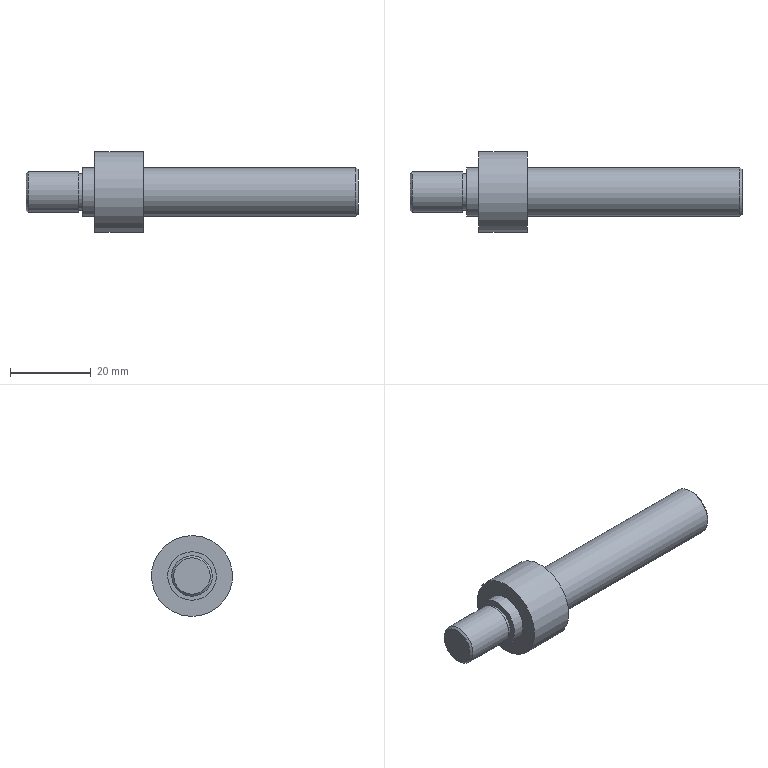Component | NX | SPINDLE | 1 solid | 13 faces | box 82 x 20 x 20 mm | volume 11180 mm3 | plane 6 | cylinder 5 | cone 2 | commonest cylinder face diameters 12 x2 20 x1 9 x1 10 x1
STEP:
#1=CARTESIAN_POINT('',(0.,0.,0.));
#2=DIRECTION('',(0.,0.,1.));
#3=DIRECTION('',(1.,0.,0.));
#4=AXIS2_PLACEMENT_3D('',#1,#2,#3);
#5=CARTESIAN_POINT('',(33.,5.083,38.6));
#6=VERTEX_POINT('',#5);
#7=CARTESIAN_POINT('',(33.,0.,36.5));
#8=DIRECTION('',(1.,0.,0.));
#9=DIRECTION('',(0.,0.9242,0.3818));
#10=AXIS2_PLACEMENT_3D('',#7,#8,#9);
#11=CIRCLE('',#10,5.5);
#12=CARTESIAN_POINT('',(33.,-5.545,34.209));
#13=DIRECTION('',(-1.,0.,0.));
#14=DIRECTION('',(0.,0.9242,0.3818));
#15=AXIS2_PLACEMENT_3D('',#12,#13,#14);
#16=PLANE('',#15);
#17=CARTESIAN_POINT('',(11.5,-0.));
#18=CARTESIAN_POINT('',(11.5,-9.526));
#19=CARTESIAN_POINT('',(3.25,-4.763));
#20=CARTESIAN_POINT('',(-5.,-0.));
#21=CARTESIAN_POINT('',(3.25,4.763));
#22=CARTESIAN_POINT('',(11.5,9.526));
#23=CARTESIAN_POINT('',(11.5,-0.));
#24=(BOUNDED_CURVE()B_SPLINE_CURVE(2,(#17,#18,#19,#20,#21,#22,#23),.UNSPECIFIED.,.T.,.F.)B_SPLINE_CURVE_WITH_KNOTS((1,2,2,2,2,1),(-2.094,0.,2.094,4.189,6.283,8.378),.UNSPECIFIED.)CURVE()GEOMETRIC_REPRESENTATION_ITEM()RATIONAL_B_SPLINE_CURVE((1.,0.5,1.,0.5,1.,0.5,1.))REPRESENTATION_ITEM(''));
#25=(GEOMETRIC_REPRESENTATION_CONTEXT(2)PARAMETRIC_REPRESENTATION_CONTEXT()REPRESENTATION_CONTEXT('',''));
#26=DEFINITIONAL_REPRESENTATION('',(#24),#25);
#27=PCURVE('',#16,#26);
#28=CARTESIAN_POINT('',(33.,0.,36.5));
#29=DIRECTION('',(-1.,0.,0.));
#30=DIRECTION('',(0.,0.9242,0.3818));
#31=AXIS2_PLACEMENT_3D('',#28,#29,#30);
#32=CONICAL_SURFACE('',#31,5.5,0.7854);
#33=CARTESIAN_POINT('',(6.283,-0.));
#34=DIRECTION('',(-1.,0.));
#35=VECTOR('',#34,1.);
#36=LINE('',#33,#35);
#37=(GEOMETRIC_REPRESENTATION_CONTEXT(2)PARAMETRIC_REPRESENTATION_CONTEXT()REPRESENTATION_CONTEXT('',''));
#38=DEFINITIONAL_REPRESENTATION('',(#36),#37);
#39=PCURVE('',#32,#38);
#40=SURFACE_CURVE('',#11,(#27,#39),.PCURVE_S1.);
#41=EDGE_CURVE('',#6,#6,#40,.T.);
#42=ORIENTED_EDGE('',*,*,#41,.T.);
#43=EDGE_LOOP('',(#42));
#44=FACE_BOUND('',#43,.T.);
#45=ADVANCED_FACE('',(#44),#16,.F.);
#46=CARTESIAN_POINT('',(32.5,5.545,38.791));
#47=VERTEX_POINT('',#46);
#48=CARTESIAN_POINT('',(32.5,-5.545,34.209));
#49=VERTEX_POINT('',#48);
#50=CARTESIAN_POINT('',(32.5,0.,36.5));
#51=DIRECTION('',(-1.,0.,0.));
#52=DIRECTION('',(0.,0.9242,0.3818));
#53=AXIS2_PLACEMENT_3D('',#50,#51,#52);
#54=CIRCLE('',#53,6.);
#55=CARTESIAN_POINT('',(33.,0.,36.5));
#56=DIRECTION('',(1.,0.,0.));
#57=DIRECTION('',(0.,-0.9242,-0.3818));
#58=AXIS2_PLACEMENT_3D('',#55,#56,#57);
#59=CYLINDRICAL_SURFACE('',#58,6.);
#60=CARTESIAN_POINT('',(3.142,-0.5));
#61=DIRECTION('',(-1.,0.));
#62=VECTOR('',#61,1.);
#63=LINE('',#60,#62);
#64=(GEOMETRIC_REPRESENTATION_CONTEXT(2)PARAMETRIC_REPRESENTATION_CONTEXT()REPRESENTATION_CONTEXT('',''));
#65=DEFINITIONAL_REPRESENTATION('',(#63),#64);
#66=PCURVE('',#59,#65);
#67=CARTESIAN_POINT('',(0.,0.5));
#68=DIRECTION('',(1.,0.));
#69=VECTOR('',#68,1.);
#70=LINE('',#67,#69);
#71=(GEOMETRIC_REPRESENTATION_CONTEXT(2)PARAMETRIC_REPRESENTATION_CONTEXT()REPRESENTATION_CONTEXT('',''));
#72=DEFINITIONAL_REPRESENTATION('',(#70),#71);
#73=PCURVE('',#32,#72);
#74=SURFACE_CURVE('',#54,(#66,#73),.PCURVE_S1.);
#75=EDGE_CURVE('',#47,#49,#74,.T.);
#76=ORIENTED_EDGE('',*,*,#75,.T.);
#77=CARTESIAN_POINT('',(-20.,-5.545,34.209));
#78=VERTEX_POINT('',#77);
#79=CARTESIAN_POINT('',(-20.,-5.545,34.209));
#80=CARTESIAN_POINT('',(32.5,-5.545,34.209));
#81=B_SPLINE_CURVE_WITH_KNOTS('',1,(#79,#80),.UNSPECIFIED.,.F.,.F.,(2,2),(-53.,-0.5),.PIECEWISE_BEZIER_KNOTS.);
#82=CARTESIAN_POINT('',(0.,0.));
#83=DIRECTION('',(0.,1.));
#84=VECTOR('',#83,1.);
#85=LINE('',#82,#84);
#86=(GEOMETRIC_REPRESENTATION_CONTEXT(2)PARAMETRIC_REPRESENTATION_CONTEXT()REPRESENTATION_CONTEXT('',''));
#87=DEFINITIONAL_REPRESENTATION('',(#85),#86);
#88=PCURVE('',#59,#87);
#89=CARTESIAN_POINT('',(6.283,0.));
#90=DIRECTION('',(0.,1.));
#91=VECTOR('',#90,1.);
#92=LINE('',#89,#91);
#93=(GEOMETRIC_REPRESENTATION_CONTEXT(2)PARAMETRIC_REPRESENTATION_CONTEXT()REPRESENTATION_CONTEXT('',''));
#94=DEFINITIONAL_REPRESENTATION('',(#92),#93);
#95=PCURVE('',#59,#94);
#96=SEAM_CURVE('',#81,(#88,#95),.PCURVE_S1.);
#97=EDGE_CURVE('',#78,#49,#96,.T.);
#98=ORIENTED_EDGE('',*,*,#97,.F.);
#99=CARTESIAN_POINT('',(-20.,0.,36.5));
#100=DIRECTION('',(1.,0.,0.));
#101=DIRECTION('',(0.,-0.9242,-0.3818));
#102=AXIS2_PLACEMENT_3D('',#99,#100,#101);
#103=CIRCLE('',#102,6.);
#104=CARTESIAN_POINT('',(0.,-53.));
#105=DIRECTION('',(1.,0.));
#106=VECTOR('',#105,1.);
#107=LINE('',#104,#106);
#108=(GEOMETRIC_REPRESENTATION_CONTEXT(2)PARAMETRIC_REPRESENTATION_CONTEXT()REPRESENTATION_CONTEXT('',''));
#109=DEFINITIONAL_REPRESENTATION('',(#107),#108);
#110=PCURVE('',#59,#109);
#111=CARTESIAN_POINT('',(-20.,-9.242,32.682));
#112=DIRECTION('',(-1.,0.,0.));
#113=DIRECTION('',(0.,0.9242,0.3818));
#114=AXIS2_PLACEMENT_3D('',#111,#112,#113);
#115=PLANE('',#114);
#116=CARTESIAN_POINT('',(4.,0.));
#117=CARTESIAN_POINT('',(4.,10.392));
#118=CARTESIAN_POINT('',(13.,5.196));
#119=CARTESIAN_POINT('',(22.,0.));
#120=CARTESIAN_POINT('',(13.,-5.196));
#121=CARTESIAN_POINT('',(4.,-10.392));
#122=CARTESIAN_POINT('',(4.,0.));
#123=(BOUNDED_CURVE()B_SPLINE_CURVE(2,(#116,#117,#118,#119,#120,#121,#122),.UNSPECIFIED.,.T.,.F.)B_SPLINE_CURVE_WITH_KNOTS((1,2,2,2,2,1),(-2.094,0.,2.094,4.189,6.283,8.378),.UNSPECIFIED.)CURVE()GEOMETRIC_REPRESENTATION_ITEM()RATIONAL_B_SPLINE_CURVE((1.,0.5,1.,0.5,1.,0.5,1.))REPRESENTATION_ITEM(''));
#124=(GEOMETRIC_REPRESENTATION_CONTEXT(2)PARAMETRIC_REPRESENTATION_CONTEXT()REPRESENTATION_CONTEXT('',''));
#125=DEFINITIONAL_REPRESENTATION('',(#123),#124);
#126=PCURVE('',#115,#125);
#127=SURFACE_CURVE('',#103,(#110,#126),.PCURVE_S1.);
#128=EDGE_CURVE('',#78,#78,#127,.T.);
#129=ORIENTED_EDGE('',*,*,#128,.T.);
#130=ORIENTED_EDGE('',*,*,#97,.T.);
#131=CARTESIAN_POINT('',(32.5,0.,36.5));
#132=DIRECTION('',(-1.,0.,0.));
#133=DIRECTION('',(0.,0.9242,0.3818));
#134=AXIS2_PLACEMENT_3D('',#131,#132,#133);
#135=CIRCLE('',#134,6.);
#136=CARTESIAN_POINT('',(9.425,-0.5));
#137=DIRECTION('',(-1.,0.));
#138=VECTOR('',#137,1.);
#139=LINE('',#136,#138);
#140=(GEOMETRIC_REPRESENTATION_CONTEXT(2)PARAMETRIC_REPRESENTATION_CONTEXT()REPRESENTATION_CONTEXT('',''));
#141=DEFINITIONAL_REPRESENTATION('',(#139),#140);
#142=PCURVE('',#59,#141);
#143=CARTESIAN_POINT('',(0.,0.5));
#144=DIRECTION('',(1.,-0.));
#145=VECTOR('',#144,1.);
#146=LINE('',#143,#145);
#147=(GEOMETRIC_REPRESENTATION_CONTEXT(2)PARAMETRIC_REPRESENTATION_CONTEXT()REPRESENTATION_CONTEXT('',''));
#148=DEFINITIONAL_REPRESENTATION('',(#146),#147);
#149=PCURVE('',#32,#148);
#150=SURFACE_CURVE('',#135,(#142,#149),.PCURVE_S1.);
#151=EDGE_CURVE('',#49,#47,#150,.T.);
#152=ORIENTED_EDGE('',*,*,#151,.T.);
#153=EDGE_LOOP('',(#76,#98,#129,#130,#152));
#154=FACE_BOUND('',#153,.T.);
#155=ADVANCED_FACE('',(#154),#59,.T.);
#156=ORIENTED_EDGE('',*,*,#128,.F.);
#157=EDGE_LOOP('',(#156));
#158=FACE_BOUND('',#157,.T.);
#159=CARTESIAN_POINT('',(-20.,-9.242,32.682));
#160=VERTEX_POINT('',#159);
#161=CARTESIAN_POINT('',(-20.,0.,36.5));
#162=DIRECTION('',(1.,0.,0.));
#163=DIRECTION('',(0.,-0.9242,-0.3818));
#164=AXIS2_PLACEMENT_3D('',#161,#162,#163);
#165=CIRCLE('',#164,10.);
#166=CARTESIAN_POINT('',(-0.,0.));
#167=CARTESIAN_POINT('',(-0.,17.321));
#168=CARTESIAN_POINT('',(15.,8.66));
#169=CARTESIAN_POINT('',(30.,0.));
#170=CARTESIAN_POINT('',(15.,-8.66));
#171=CARTESIAN_POINT('',(0.,-17.321));
#172=CARTESIAN_POINT('',(-0.,0.));
#173=(BOUNDED_CURVE()B_SPLINE_CURVE(2,(#166,#167,#168,#169,#170,#171,#172),.UNSPECIFIED.,.T.,.F.)B_SPLINE_CURVE_WITH_KNOTS((1,2,2,2,2,1),(-2.094,0.,2.094,4.189,6.283,8.378),.UNSPECIFIED.)CURVE()GEOMETRIC_REPRESENTATION_ITEM()RATIONAL_B_SPLINE_CURVE((1.,0.5,1.,0.5,1.,0.5,1.))REPRESENTATION_ITEM(''));
#174=(GEOMETRIC_REPRESENTATION_CONTEXT(2)PARAMETRIC_REPRESENTATION_CONTEXT()REPRESENTATION_CONTEXT('',''));
#175=DEFINITIONAL_REPRESENTATION('',(#173),#174);
#176=PCURVE('',#115,#175);
#177=CARTESIAN_POINT('',(33.,0.,36.5));
#178=DIRECTION('',(1.,0.,0.));
#179=DIRECTION('',(0.,-0.9242,-0.3818));
#180=AXIS2_PLACEMENT_3D('',#177,#178,#179);
#181=CYLINDRICAL_SURFACE('',#180,10.);
#182=CARTESIAN_POINT('',(0.,-53.));
#183=DIRECTION('',(1.,0.));
#184=VECTOR('',#183,1.);
#185=LINE('',#182,#184);
#186=(GEOMETRIC_REPRESENTATION_CONTEXT(2)PARAMETRIC_REPRESENTATION_CONTEXT()REPRESENTATION_CONTEXT('',''));
#187=DEFINITIONAL_REPRESENTATION('',(#185),#186);
#188=PCURVE('',#181,#187);
#189=SURFACE_CURVE('',#165,(#176,#188),.PCURVE_S1.);
#190=EDGE_CURVE('',#160,#160,#189,.T.);
#191=ORIENTED_EDGE('',*,*,#190,.T.);
#192=EDGE_LOOP('',(#191));
#193=FACE_BOUND('',#192,.T.);
#194=ADVANCED_FACE('',(#158,#193),#115,.F.);
#195=ORIENTED_EDGE('',*,*,#190,.F.);
#196=CARTESIAN_POINT('',(-32.,-9.242,32.682));
#197=VERTEX_POINT('',#196);
#198=CARTESIAN_POINT('',(-32.,-9.242,32.682));
#199=CARTESIAN_POINT('',(-20.,-9.242,32.682));
#200=B_SPLINE_CURVE_WITH_KNOTS('',1,(#198,#199),.UNSPECIFIED.,.F.,.F.,(2,2),(-65.,-53.),.PIECEWISE_BEZIER_KNOTS.);
#201=CARTESIAN_POINT('',(0.,0.));
#202=DIRECTION('',(0.,1.));
#203=VECTOR('',#202,1.);
#204=LINE('',#201,#203);
#205=(GEOMETRIC_REPRESENTATION_CONTEXT(2)PARAMETRIC_REPRESENTATION_CONTEXT()REPRESENTATION_CONTEXT('',''));
#206=DEFINITIONAL_REPRESENTATION('',(#204),#205);
#207=PCURVE('',#181,#206);
#208=CARTESIAN_POINT('',(6.283,0.));
#209=DIRECTION('',(0.,1.));
#210=VECTOR('',#209,1.);
#211=LINE('',#208,#210);
#212=(GEOMETRIC_REPRESENTATION_CONTEXT(2)PARAMETRIC_REPRESENTATION_CONTEXT()REPRESENTATION_CONTEXT('',''));
#213=DEFINITIONAL_REPRESENTATION('',(#211),#212);
#214=PCURVE('',#181,#213);
#215=SEAM_CURVE('',#200,(#207,#214),.PCURVE_S1.);
#216=EDGE_CURVE('',#197,#160,#215,.T.);
#217=ORIENTED_EDGE('',*,*,#216,.F.);
#218=CARTESIAN_POINT('',(-32.,0.,36.5));
#219=DIRECTION('',(1.,0.,0.));
#220=DIRECTION('',(0.,-0.9242,-0.3818));
#221=AXIS2_PLACEMENT_3D('',#218,#219,#220);
#222=CIRCLE('',#221,10.);
#223=CARTESIAN_POINT('',(0.,-65.));
#224=DIRECTION('',(1.,0.));
#225=VECTOR('',#224,1.);
#226=LINE('',#223,#225);
#227=(GEOMETRIC_REPRESENTATION_CONTEXT(2)PARAMETRIC_REPRESENTATION_CONTEXT()REPRESENTATION_CONTEXT('',''));
#228=DEFINITIONAL_REPRESENTATION('',(#226),#227);
#229=PCURVE('',#181,#228);
#230=CARTESIAN_POINT('',(-32.,-5.545,34.209));
#231=DIRECTION('',(1.,0.,0.));
#232=DIRECTION('',(0.,-0.9242,-0.3818));
#233=AXIS2_PLACEMENT_3D('',#230,#231,#232);
#234=PLANE('',#233);
#235=CARTESIAN_POINT('',(-6.,-0.));
#236=DIRECTION('',(1.,0.));
#237=AXIS2_PLACEMENT_2D('',#235,#236);
#238=CIRCLE('',#237,10.);
#239=(GEOMETRIC_REPRESENTATION_CONTEXT(2)PARAMETRIC_REPRESENTATION_CONTEXT()REPRESENTATION_CONTEXT('',''));
#240=DEFINITIONAL_REPRESENTATION('',(#238),#239);
#241=PCURVE('',#234,#240);
#242=SURFACE_CURVE('',#222,(#229,#241),.PCURVE_S1.);
#243=EDGE_CURVE('',#197,#197,#242,.T.);
#244=ORIENTED_EDGE('',*,*,#243,.T.);
#245=ORIENTED_EDGE('',*,*,#216,.T.);
#246=EDGE_LOOP('',(#195,#217,#244,#245));
#247=FACE_BOUND('',#246,.T.);
#248=ADVANCED_FACE('',(#247),#181,.T.);
#249=ORIENTED_EDGE('',*,*,#243,.F.);
#250=EDGE_LOOP('',(#249));
#251=FACE_BOUND('',#250,.T.);
#252=CARTESIAN_POINT('',(-32.,-5.545,34.209));
#253=VERTEX_POINT('',#252);
#254=CARTESIAN_POINT('',(-32.,0.,36.5));
#255=DIRECTION('',(1.,0.,0.));
#256=DIRECTION('',(0.,-0.9242,-0.3818));
#257=AXIS2_PLACEMENT_3D('',#254,#255,#256);
#258=CIRCLE('',#257,6.);
#259=CARTESIAN_POINT('',(-6.,-0.));
#260=DIRECTION('',(1.,0.));
#261=AXIS2_PLACEMENT_2D('',#259,#260);
#262=CIRCLE('',#261,6.);
#263=(GEOMETRIC_REPRESENTATION_CONTEXT(2)PARAMETRIC_REPRESENTATION_CONTEXT()REPRESENTATION_CONTEXT('',''));
#264=DEFINITIONAL_REPRESENTATION('',(#262),#263);
#265=PCURVE('',#234,#264);
#266=CARTESIAN_POINT('',(33.,0.,36.5));
#267=DIRECTION('',(1.,0.,0.));
#268=DIRECTION('',(0.,-0.9242,-0.3818));
#269=AXIS2_PLACEMENT_3D('',#266,#267,#268);
#270=CYLINDRICAL_SURFACE('',#269,6.);
#271=CARTESIAN_POINT('',(0.,-65.));
#272=DIRECTION('',(1.,0.));
#273=VECTOR('',#272,1.);
#274=LINE('',#271,#273);
#275=(GEOMETRIC_REPRESENTATION_CONTEXT(2)PARAMETRIC_REPRESENTATION_CONTEXT()REPRESENTATION_CONTEXT('',''));
#276=DEFINITIONAL_REPRESENTATION('',(#274),#275);
#277=PCURVE('',#270,#276);
#278=SURFACE_CURVE('',#258,(#265,#277),.PCURVE_S1.);
#279=EDGE_CURVE('',#253,#253,#278,.T.);
#280=ORIENTED_EDGE('',*,*,#279,.T.);
#281=EDGE_LOOP('',(#280));
#282=FACE_BOUND('',#281,.T.);
#283=ADVANCED_FACE('',(#251,#282),#234,.F.);
#284=ORIENTED_EDGE('',*,*,#279,.F.);
#285=CARTESIAN_POINT('',(-35.,-5.545,34.209));
#286=VERTEX_POINT('',#285);
#287=CARTESIAN_POINT('',(-35.,-5.545,34.209));
#288=CARTESIAN_POINT('',(-32.,-5.545,34.209));
#289=B_SPLINE_CURVE_WITH_KNOTS('',1,(#287,#288),.UNSPECIFIED.,.F.,.F.,(2,2),(-68.,-65.),.PIECEWISE_BEZIER_KNOTS.);
#290=CARTESIAN_POINT('',(0.,0.));
#291=DIRECTION('',(0.,1.));
#292=VECTOR('',#291,1.);
#293=LINE('',#290,#292);
#294=(GEOMETRIC_REPRESENTATION_CONTEXT(2)PARAMETRIC_REPRESENTATION_CONTEXT()REPRESENTATION_CONTEXT('',''));
#295=DEFINITIONAL_REPRESENTATION('',(#293),#294);
#296=PCURVE('',#270,#295);
#297=CARTESIAN_POINT('',(6.283,0.));
#298=DIRECTION('',(0.,1.));
#299=VECTOR('',#298,1.);
#300=LINE('',#297,#299);
#301=(GEOMETRIC_REPRESENTATION_CONTEXT(2)PARAMETRIC_REPRESENTATION_CONTEXT()REPRESENTATION_CONTEXT('',''));
#302=DEFINITIONAL_REPRESENTATION('',(#300),#301);
#303=PCURVE('',#270,#302);
#304=SEAM_CURVE('',#289,(#296,#303),.PCURVE_S1.);
#305=EDGE_CURVE('',#286,#253,#304,.T.);
#306=ORIENTED_EDGE('',*,*,#305,.F.);
#307=CARTESIAN_POINT('',(-35.,0.,36.5));
#308=DIRECTION('',(1.,0.,0.));
#309=DIRECTION('',(0.,-0.9242,-0.3818));
#310=AXIS2_PLACEMENT_3D('',#307,#308,#309);
#311=CIRCLE('',#310,6.);
#312=CARTESIAN_POINT('',(0.,-68.));
#313=DIRECTION('',(1.,0.));
#314=VECTOR('',#313,1.);
#315=LINE('',#312,#314);
#316=(GEOMETRIC_REPRESENTATION_CONTEXT(2)PARAMETRIC_REPRESENTATION_CONTEXT()REPRESENTATION_CONTEXT('',''));
#317=DEFINITIONAL_REPRESENTATION('',(#315),#316);
#318=PCURVE('',#270,#317);
#319=CARTESIAN_POINT('',(-35.,-4.159,34.782));
#320=DIRECTION('',(1.,0.,0.));
#321=DIRECTION('',(0.,-0.9242,-0.3818));
#322=AXIS2_PLACEMENT_3D('',#319,#320,#321);
#323=PLANE('',#322);
#324=CARTESIAN_POINT('',(-4.5,-0.));
#325=DIRECTION('',(1.,0.));
#326=AXIS2_PLACEMENT_2D('',#324,#325);
#327=CIRCLE('',#326,6.);
#328=(GEOMETRIC_REPRESENTATION_CONTEXT(2)PARAMETRIC_REPRESENTATION_CONTEXT()REPRESENTATION_CONTEXT('',''));
#329=DEFINITIONAL_REPRESENTATION('',(#327),#328);
#330=PCURVE('',#323,#329);
#331=SURFACE_CURVE('',#311,(#318,#330),.PCURVE_S1.);
#332=EDGE_CURVE('',#286,#286,#331,.T.);
#333=ORIENTED_EDGE('',*,*,#332,.T.);
#334=ORIENTED_EDGE('',*,*,#305,.T.);
#335=EDGE_LOOP('',(#284,#306,#333,#334));
#336=FACE_BOUND('',#335,.T.);
#337=ADVANCED_FACE('',(#336),#270,.T.);
#338=ORIENTED_EDGE('',*,*,#332,.F.);
#339=EDGE_LOOP('',(#338));
#340=FACE_BOUND('',#339,.T.);
#341=CARTESIAN_POINT('',(-35.,-4.159,34.782));
#342=VERTEX_POINT('',#341);
#343=CARTESIAN_POINT('',(-35.,0.,36.5));
#344=DIRECTION('',(1.,0.,0.));
#345=DIRECTION('',(0.,-0.9242,-0.3818));
#346=AXIS2_PLACEMENT_3D('',#343,#344,#345);
#347=CIRCLE('',#346,4.5);
#348=CARTESIAN_POINT('',(-4.5,-0.));
#349=DIRECTION('',(1.,0.));
#350=AXIS2_PLACEMENT_2D('',#348,#349);
#351=CIRCLE('',#350,4.5);
#352=(GEOMETRIC_REPRESENTATION_CONTEXT(2)PARAMETRIC_REPRESENTATION_CONTEXT()REPRESENTATION_CONTEXT('',''));
#353=DEFINITIONAL_REPRESENTATION('',(#351),#352);
#354=PCURVE('',#323,#353);
#355=CARTESIAN_POINT('',(33.,0.,36.5));
#356=DIRECTION('',(1.,0.,0.));
#357=DIRECTION('',(0.,-0.9242,-0.3818));
#358=AXIS2_PLACEMENT_3D('',#355,#356,#357);
#359=CYLINDRICAL_SURFACE('',#358,4.5);
#360=CARTESIAN_POINT('',(0.,-68.));
#361=DIRECTION('',(1.,0.));
#362=VECTOR('',#361,1.);
#363=LINE('',#360,#362);
#364=(GEOMETRIC_REPRESENTATION_CONTEXT(2)PARAMETRIC_REPRESENTATION_CONTEXT()REPRESENTATION_CONTEXT('',''));
#365=DEFINITIONAL_REPRESENTATION('',(#363),#364);
#366=PCURVE('',#359,#365);
#367=SURFACE_CURVE('',#347,(#354,#366),.PCURVE_S1.);
#368=EDGE_CURVE('',#342,#342,#367,.T.);
#369=ORIENTED_EDGE('',*,*,#368,.T.);
#370=EDGE_LOOP('',(#369));
#371=FACE_BOUND('',#370,.T.);
#372=ADVANCED_FACE('',(#340,#371),#323,.F.);
#373=ORIENTED_EDGE('',*,*,#368,.F.);
#374=CARTESIAN_POINT('',(-36.,-4.159,34.782));
#375=VERTEX_POINT('',#374);
#376=CARTESIAN_POINT('',(-36.,-4.159,34.782));
#377=CARTESIAN_POINT('',(-35.,-4.159,34.782));
#378=B_SPLINE_CURVE_WITH_KNOTS('',1,(#376,#377),.UNSPECIFIED.,.F.,.F.,(2,2),(-69.,-68.),.PIECEWISE_BEZIER_KNOTS.);
#379=CARTESIAN_POINT('',(0.,0.));
#380=DIRECTION('',(0.,1.));
#381=VECTOR('',#380,1.);
#382=LINE('',#379,#381);
#383=(GEOMETRIC_REPRESENTATION_CONTEXT(2)PARAMETRIC_REPRESENTATION_CONTEXT()REPRESENTATION_CONTEXT('',''));
#384=DEFINITIONAL_REPRESENTATION('',(#382),#383);
#385=PCURVE('',#359,#384);
#386=CARTESIAN_POINT('',(6.283,0.));
#387=DIRECTION('',(0.,1.));
#388=VECTOR('',#387,1.);
#389=LINE('',#386,#388);
#390=(GEOMETRIC_REPRESENTATION_CONTEXT(2)PARAMETRIC_REPRESENTATION_CONTEXT()REPRESENTATION_CONTEXT('',''));
#391=DEFINITIONAL_REPRESENTATION('',(#389),#390);
#392=PCURVE('',#359,#391);
#393=SEAM_CURVE('',#378,(#385,#392),.PCURVE_S1.);
#394=EDGE_CURVE('',#375,#342,#393,.T.);
#395=ORIENTED_EDGE('',*,*,#394,.F.);
#396=CARTESIAN_POINT('',(-36.,0.,36.5));
#397=DIRECTION('',(1.,0.,0.));
#398=DIRECTION('',(0.,-0.9242,-0.3818));
#399=AXIS2_PLACEMENT_3D('',#396,#397,#398);
#400=CIRCLE('',#399,4.5);
#401=CARTESIAN_POINT('',(0.,-69.));
#402=DIRECTION('',(1.,0.));
#403=VECTOR('',#402,1.);
#404=LINE('',#401,#403);
#405=(GEOMETRIC_REPRESENTATION_CONTEXT(2)PARAMETRIC_REPRESENTATION_CONTEXT()REPRESENTATION_CONTEXT('',''));
#406=DEFINITIONAL_REPRESENTATION('',(#404),#405);
#407=PCURVE('',#359,#406);
#408=CARTESIAN_POINT('',(-36.,-4.621,34.591));
#409=DIRECTION('',(-1.,0.,0.));
#410=DIRECTION('',(0.,0.9242,0.3818));
#411=AXIS2_PLACEMENT_3D('',#408,#409,#410);
#412=PLANE('',#411);
#413=CARTESIAN_POINT('',(0.5,-0.));
#414=CARTESIAN_POINT('',(0.5,7.794));
#415=CARTESIAN_POINT('',(7.25,3.897));
#416=CARTESIAN_POINT('',(14.,-0.));
#417=CARTESIAN_POINT('',(7.25,-3.897));
#418=CARTESIAN_POINT('',(0.5,-7.794));
#419=CARTESIAN_POINT('',(0.5,-0.));
#420=(BOUNDED_CURVE()B_SPLINE_CURVE(2,(#413,#414,#415,#416,#417,#418,#419),.UNSPECIFIED.,.T.,.F.)B_SPLINE_CURVE_WITH_KNOTS((1,2,2,2,2,1),(-2.094,0.,2.094,4.189,6.283,8.378),.UNSPECIFIED.)CURVE()GEOMETRIC_REPRESENTATION_ITEM()RATIONAL_B_SPLINE_CURVE((1.,0.5,1.,0.5,1.,0.5,1.))REPRESENTATION_ITEM(''));
#421=(GEOMETRIC_REPRESENTATION_CONTEXT(2)PARAMETRIC_REPRESENTATION_CONTEXT()REPRESENTATION_CONTEXT('',''));
#422=DEFINITIONAL_REPRESENTATION('',(#420),#421);
#423=PCURVE('',#412,#422);
#424=SURFACE_CURVE('',#400,(#407,#423),.PCURVE_S1.);
#425=EDGE_CURVE('',#375,#375,#424,.T.);
#426=ORIENTED_EDGE('',*,*,#425,.T.);
#427=ORIENTED_EDGE('',*,*,#394,.T.);
#428=EDGE_LOOP('',(#373,#395,#426,#427));
#429=FACE_BOUND('',#428,.T.);
#430=ADVANCED_FACE('',(#429),#359,.T.);
#431=ORIENTED_EDGE('',*,*,#425,.F.);
#432=EDGE_LOOP('',(#431));
#433=FACE_BOUND('',#432,.T.);
#434=CARTESIAN_POINT('',(-36.,-4.621,34.591));
#435=VERTEX_POINT('',#434);
#436=CARTESIAN_POINT('',(-36.,0.,36.5));
#437=DIRECTION('',(1.,0.,0.));
#438=DIRECTION('',(0.,-0.9242,-0.3818));
#439=AXIS2_PLACEMENT_3D('',#436,#437,#438);
#440=CIRCLE('',#439,5.);
#441=CARTESIAN_POINT('',(0.,-0.));
#442=CARTESIAN_POINT('',(0.,8.66));
#443=CARTESIAN_POINT('',(7.5,4.33));
#444=CARTESIAN_POINT('',(15.,-0.));
#445=CARTESIAN_POINT('',(7.5,-4.33));
#446=CARTESIAN_POINT('',(0.,-8.66));
#447=CARTESIAN_POINT('',(0.,-0.));
#448=(BOUNDED_CURVE()B_SPLINE_CURVE(2,(#441,#442,#443,#444,#445,#446,#447),.UNSPECIFIED.,.T.,.F.)B_SPLINE_CURVE_WITH_KNOTS((1,2,2,2,2,1),(-2.094,0.,2.094,4.189,6.283,8.378),.UNSPECIFIED.)CURVE()GEOMETRIC_REPRESENTATION_ITEM()RATIONAL_B_SPLINE_CURVE((1.,0.5,1.,0.5,1.,0.5,1.))REPRESENTATION_ITEM(''));
#449=(GEOMETRIC_REPRESENTATION_CONTEXT(2)PARAMETRIC_REPRESENTATION_CONTEXT()REPRESENTATION_CONTEXT('',''));
#450=DEFINITIONAL_REPRESENTATION('',(#448),#449);
#451=PCURVE('',#412,#450);
#452=CARTESIAN_POINT('',(33.,0.,36.5));
#453=DIRECTION('',(1.,0.,0.));
#454=DIRECTION('',(0.,-0.9242,-0.3818));
#455=AXIS2_PLACEMENT_3D('',#452,#453,#454);
#456=CYLINDRICAL_SURFACE('',#455,5.);
#457=CARTESIAN_POINT('',(0.,-69.));
#458=DIRECTION('',(1.,0.));
#459=VECTOR('',#458,1.);
#460=LINE('',#457,#459);
#461=(GEOMETRIC_REPRESENTATION_CONTEXT(2)PARAMETRIC_REPRESENTATION_CONTEXT()REPRESENTATION_CONTEXT('',''));
#462=DEFINITIONAL_REPRESENTATION('',(#460),#461);
#463=PCURVE('',#456,#462);
#464=SURFACE_CURVE('',#440,(#451,#463),.PCURVE_S1.);
#465=EDGE_CURVE('',#435,#435,#464,.T.);
#466=ORIENTED_EDGE('',*,*,#465,.T.);
#467=EDGE_LOOP('',(#466));
#468=FACE_BOUND('',#467,.T.);
#469=ADVANCED_FACE('',(#433,#468),#412,.F.);
#470=CARTESIAN_POINT('',(-48.5,-4.621,34.591));
#471=VERTEX_POINT('',#470);
#472=CARTESIAN_POINT('',(-48.5,0.,36.5));
#473=DIRECTION('',(1.,0.,0.));
#474=DIRECTION('',(0.,-0.9242,-0.3818));
#475=AXIS2_PLACEMENT_3D('',#472,#473,#474);
#476=CIRCLE('',#475,5.);
#477=CARTESIAN_POINT('',(0.,-81.5));
#478=DIRECTION('',(1.,0.));
#479=VECTOR('',#478,1.);
#480=LINE('',#477,#479);
#481=(GEOMETRIC_REPRESENTATION_CONTEXT(2)PARAMETRIC_REPRESENTATION_CONTEXT()REPRESENTATION_CONTEXT('',''));
#482=DEFINITIONAL_REPRESENTATION('',(#480),#481);
#483=PCURVE('',#456,#482);
#484=CARTESIAN_POINT('',(-48.5,0.,36.5));
#485=DIRECTION('',(1.,0.,0.));
#486=DIRECTION('',(0.,-0.9242,-0.3818));
#487=AXIS2_PLACEMENT_3D('',#484,#485,#486);
#488=CONICAL_SURFACE('',#487,5.,0.7854);
#489=CARTESIAN_POINT('',(0.,0.));
#490=DIRECTION('',(1.,-0.));
#491=VECTOR('',#490,1.);
#492=LINE('',#489,#491);
#493=(GEOMETRIC_REPRESENTATION_CONTEXT(2)PARAMETRIC_REPRESENTATION_CONTEXT()REPRESENTATION_CONTEXT('',''));
#494=DEFINITIONAL_REPRESENTATION('',(#492),#493);
#495=PCURVE('',#488,#494);
#496=SURFACE_CURVE('',#476,(#483,#495),.PCURVE_S1.);
#497=EDGE_CURVE('',#471,#471,#496,.T.);
#498=ORIENTED_EDGE('',*,*,#497,.T.);
#499=CARTESIAN_POINT('',(-48.5,-4.621,34.591));
#500=CARTESIAN_POINT('',(-36.,-4.621,34.591));
#501=B_SPLINE_CURVE_WITH_KNOTS('',1,(#499,#500),.UNSPECIFIED.,.F.,.F.,(2,2),(-81.5,-69.),.PIECEWISE_BEZIER_KNOTS.);
#502=CARTESIAN_POINT('',(6.283,0.));
#503=DIRECTION('',(0.,1.));
#504=VECTOR('',#503,1.);
#505=LINE('',#502,#504);
#506=(GEOMETRIC_REPRESENTATION_CONTEXT(2)PARAMETRIC_REPRESENTATION_CONTEXT()REPRESENTATION_CONTEXT('',''));
#507=DEFINITIONAL_REPRESENTATION('',(#505),#506);
#508=PCURVE('',#456,#507);
#509=CARTESIAN_POINT('',(0.,0.));
#510=DIRECTION('',(0.,1.));
#511=VECTOR('',#510,1.);
#512=LINE('',#509,#511);
#513=(GEOMETRIC_REPRESENTATION_CONTEXT(2)PARAMETRIC_REPRESENTATION_CONTEXT()REPRESENTATION_CONTEXT('',''));
#514=DEFINITIONAL_REPRESENTATION('',(#512),#513);
#515=PCURVE('',#456,#514);
#516=SEAM_CURVE('',#501,(#508,#515),.PCURVE_S1.);
#517=EDGE_CURVE('',#471,#435,#516,.T.);
#518=ORIENTED_EDGE('',*,*,#517,.T.);
#519=ORIENTED_EDGE('',*,*,#465,.F.);
#520=ORIENTED_EDGE('',*,*,#517,.F.);
#521=EDGE_LOOP('',(#498,#518,#519,#520));
#522=FACE_BOUND('',#521,.T.);
#523=ADVANCED_FACE('',(#522),#456,.T.);
#524=CARTESIAN_POINT('',(-49.,-4.159,34.782));
#525=VERTEX_POINT('',#524);
#526=CARTESIAN_POINT('',(-49.,0.,36.5));
#527=DIRECTION('',(-1.,0.,0.));
#528=DIRECTION('',(0.,-0.9242,-0.3818));
#529=AXIS2_PLACEMENT_3D('',#526,#527,#528);
#530=CIRCLE('',#529,4.5);
#531=CARTESIAN_POINT('',(-49.,0.,36.5));
#532=DIRECTION('',(1.,0.,0.));
#533=DIRECTION('',(0.,-0.9242,-0.3818));
#534=AXIS2_PLACEMENT_3D('',#531,#532,#533);
#535=PLANE('',#534);
#536=CARTESIAN_POINT('',(4.5,0.));
#537=CARTESIAN_POINT('',(4.5,-7.794));
#538=CARTESIAN_POINT('',(-2.25,-3.897));
#539=CARTESIAN_POINT('',(-9.,-0.));
#540=CARTESIAN_POINT('',(-2.25,3.897));
#541=CARTESIAN_POINT('',(4.5,7.794));
#542=CARTESIAN_POINT('',(4.5,0.));
#543=(BOUNDED_CURVE()B_SPLINE_CURVE(2,(#536,#537,#538,#539,#540,#541,#542),.UNSPECIFIED.,.T.,.F.)B_SPLINE_CURVE_WITH_KNOTS((1,2,2,2,2,1),(-2.094,0.,2.094,4.189,6.283,8.378),.UNSPECIFIED.)CURVE()GEOMETRIC_REPRESENTATION_ITEM()RATIONAL_B_SPLINE_CURVE((1.,0.5,1.,0.5,1.,0.5,1.))REPRESENTATION_ITEM(''));
#544=(GEOMETRIC_REPRESENTATION_CONTEXT(2)PARAMETRIC_REPRESENTATION_CONTEXT()REPRESENTATION_CONTEXT('',''));
#545=DEFINITIONAL_REPRESENTATION('',(#543),#544);
#546=PCURVE('',#535,#545);
#547=CARTESIAN_POINT('',(6.283,-0.5));
#548=DIRECTION('',(-1.,0.));
#549=VECTOR('',#548,1.);
#550=LINE('',#547,#549);
#551=(GEOMETRIC_REPRESENTATION_CONTEXT(2)PARAMETRIC_REPRESENTATION_CONTEXT()REPRESENTATION_CONTEXT('',''));
#552=DEFINITIONAL_REPRESENTATION('',(#550),#551);
#553=PCURVE('',#488,#552);
#554=SURFACE_CURVE('',#530,(#546,#553),.PCURVE_S1.);
#555=EDGE_CURVE('',#525,#525,#554,.T.);
#556=ORIENTED_EDGE('',*,*,#555,.T.);
#557=EDGE_LOOP('',(#556));
#558=FACE_BOUND('',#557,.T.);
#559=ADVANCED_FACE('',(#558),#535,.F.);
#560=ORIENTED_EDGE('',*,*,#75,.F.);
#561=CARTESIAN_POINT('',(33.,5.083,38.6));
#562=CARTESIAN_POINT('',(32.5,5.545,38.791));
#563=B_SPLINE_CURVE_WITH_KNOTS('',1,(#561,#562),.UNSPECIFIED.,.F.,.F.,(2,2),(-0.,0.7071),.PIECEWISE_BEZIER_KNOTS.);
#564=CARTESIAN_POINT('',(0.,0.));
#565=DIRECTION('',(0.,1.));
#566=VECTOR('',#565,1.);
#567=LINE('',#564,#566);
#568=(GEOMETRIC_REPRESENTATION_CONTEXT(2)PARAMETRIC_REPRESENTATION_CONTEXT()REPRESENTATION_CONTEXT('',''));
#569=DEFINITIONAL_REPRESENTATION('',(#567),#568);
#570=PCURVE('',#32,#569);
#571=CARTESIAN_POINT('',(6.283,0.));
#572=DIRECTION('',(0.,1.));
#573=VECTOR('',#572,1.);
#574=LINE('',#571,#573);
#575=(GEOMETRIC_REPRESENTATION_CONTEXT(2)PARAMETRIC_REPRESENTATION_CONTEXT()REPRESENTATION_CONTEXT('',''));
#576=DEFINITIONAL_REPRESENTATION('',(#574),#575);
#577=PCURVE('',#32,#576);
#578=SEAM_CURVE('',#563,(#570,#577),.PCURVE_S1.);
#579=EDGE_CURVE('',#6,#47,#578,.T.);
#580=ORIENTED_EDGE('',*,*,#579,.F.);
#581=ORIENTED_EDGE('',*,*,#41,.F.);
#582=ORIENTED_EDGE('',*,*,#579,.T.);
#583=ORIENTED_EDGE('',*,*,#151,.F.);
#584=EDGE_LOOP('',(#560,#580,#581,#582,#583));
#585=FACE_BOUND('',#584,.T.);
#586=ADVANCED_FACE('',(#585),#32,.T.);
#587=ORIENTED_EDGE('',*,*,#555,.F.);
#588=CARTESIAN_POINT('',(-49.,-4.159,34.782));
#589=CARTESIAN_POINT('',(-48.5,-4.621,34.591));
#590=B_SPLINE_CURVE_WITH_KNOTS('',1,(#588,#589),.UNSPECIFIED.,.F.,.F.,(2,2),(-0.7071,0.),.PIECEWISE_BEZIER_KNOTS.);
#591=CARTESIAN_POINT('',(6.283,0.));
#592=DIRECTION('',(0.,1.));
#593=VECTOR('',#592,1.);
#594=LINE('',#591,#593);
#595=(GEOMETRIC_REPRESENTATION_CONTEXT(2)PARAMETRIC_REPRESENTATION_CONTEXT()REPRESENTATION_CONTEXT('',''));
#596=DEFINITIONAL_REPRESENTATION('',(#594),#595);
#597=PCURVE('',#488,#596);
#598=CARTESIAN_POINT('',(0.,0.));
#599=DIRECTION('',(0.,1.));
#600=VECTOR('',#599,1.);
#601=LINE('',#598,#600);
#602=(GEOMETRIC_REPRESENTATION_CONTEXT(2)PARAMETRIC_REPRESENTATION_CONTEXT()REPRESENTATION_CONTEXT('',''));
#603=DEFINITIONAL_REPRESENTATION('',(#601),#602);
#604=PCURVE('',#488,#603);
#605=SEAM_CURVE('',#590,(#597,#604),.PCURVE_S1.);
#606=EDGE_CURVE('',#525,#471,#605,.T.);
#607=ORIENTED_EDGE('',*,*,#606,.T.);
#608=ORIENTED_EDGE('',*,*,#497,.F.);
#609=ORIENTED_EDGE('',*,*,#606,.F.);
#610=EDGE_LOOP('',(#587,#607,#608,#609));
#611=FACE_BOUND('',#610,.T.);
#612=ADVANCED_FACE('',(#611),#488,.T.);
#613=CLOSED_SHELL('',(#45,#155,#194,#248,#283,#337,#372,#430,#469,#523,#559,#586,#612));
#614=MANIFOLD_SOLID_BREP('',#613);
#615=(LENGTH_UNIT()NAMED_UNIT(*)SI_UNIT(.MILLI.,.METRE.));
#616=UNCERTAINTY_MEASURE_WITH_UNIT(LENGTH_MEASURE(0.00001),#615,'','');
#617=(NAMED_UNIT(*)PLANE_ANGLE_UNIT()SI_UNIT($,.RADIAN.));
#618=(NAMED_UNIT(*)SI_UNIT($,.STERADIAN.)SOLID_ANGLE_UNIT());
#619=(GEOMETRIC_REPRESENTATION_CONTEXT(3)GLOBAL_UNCERTAINTY_ASSIGNED_CONTEXT((#616))GLOBAL_UNIT_ASSIGNED_CONTEXT((#615,#617,#618))REPRESENTATION_CONTEXT('',''));
#620=ADVANCED_BREP_SHAPE_REPRESENTATION('',(#4,#614),#619);